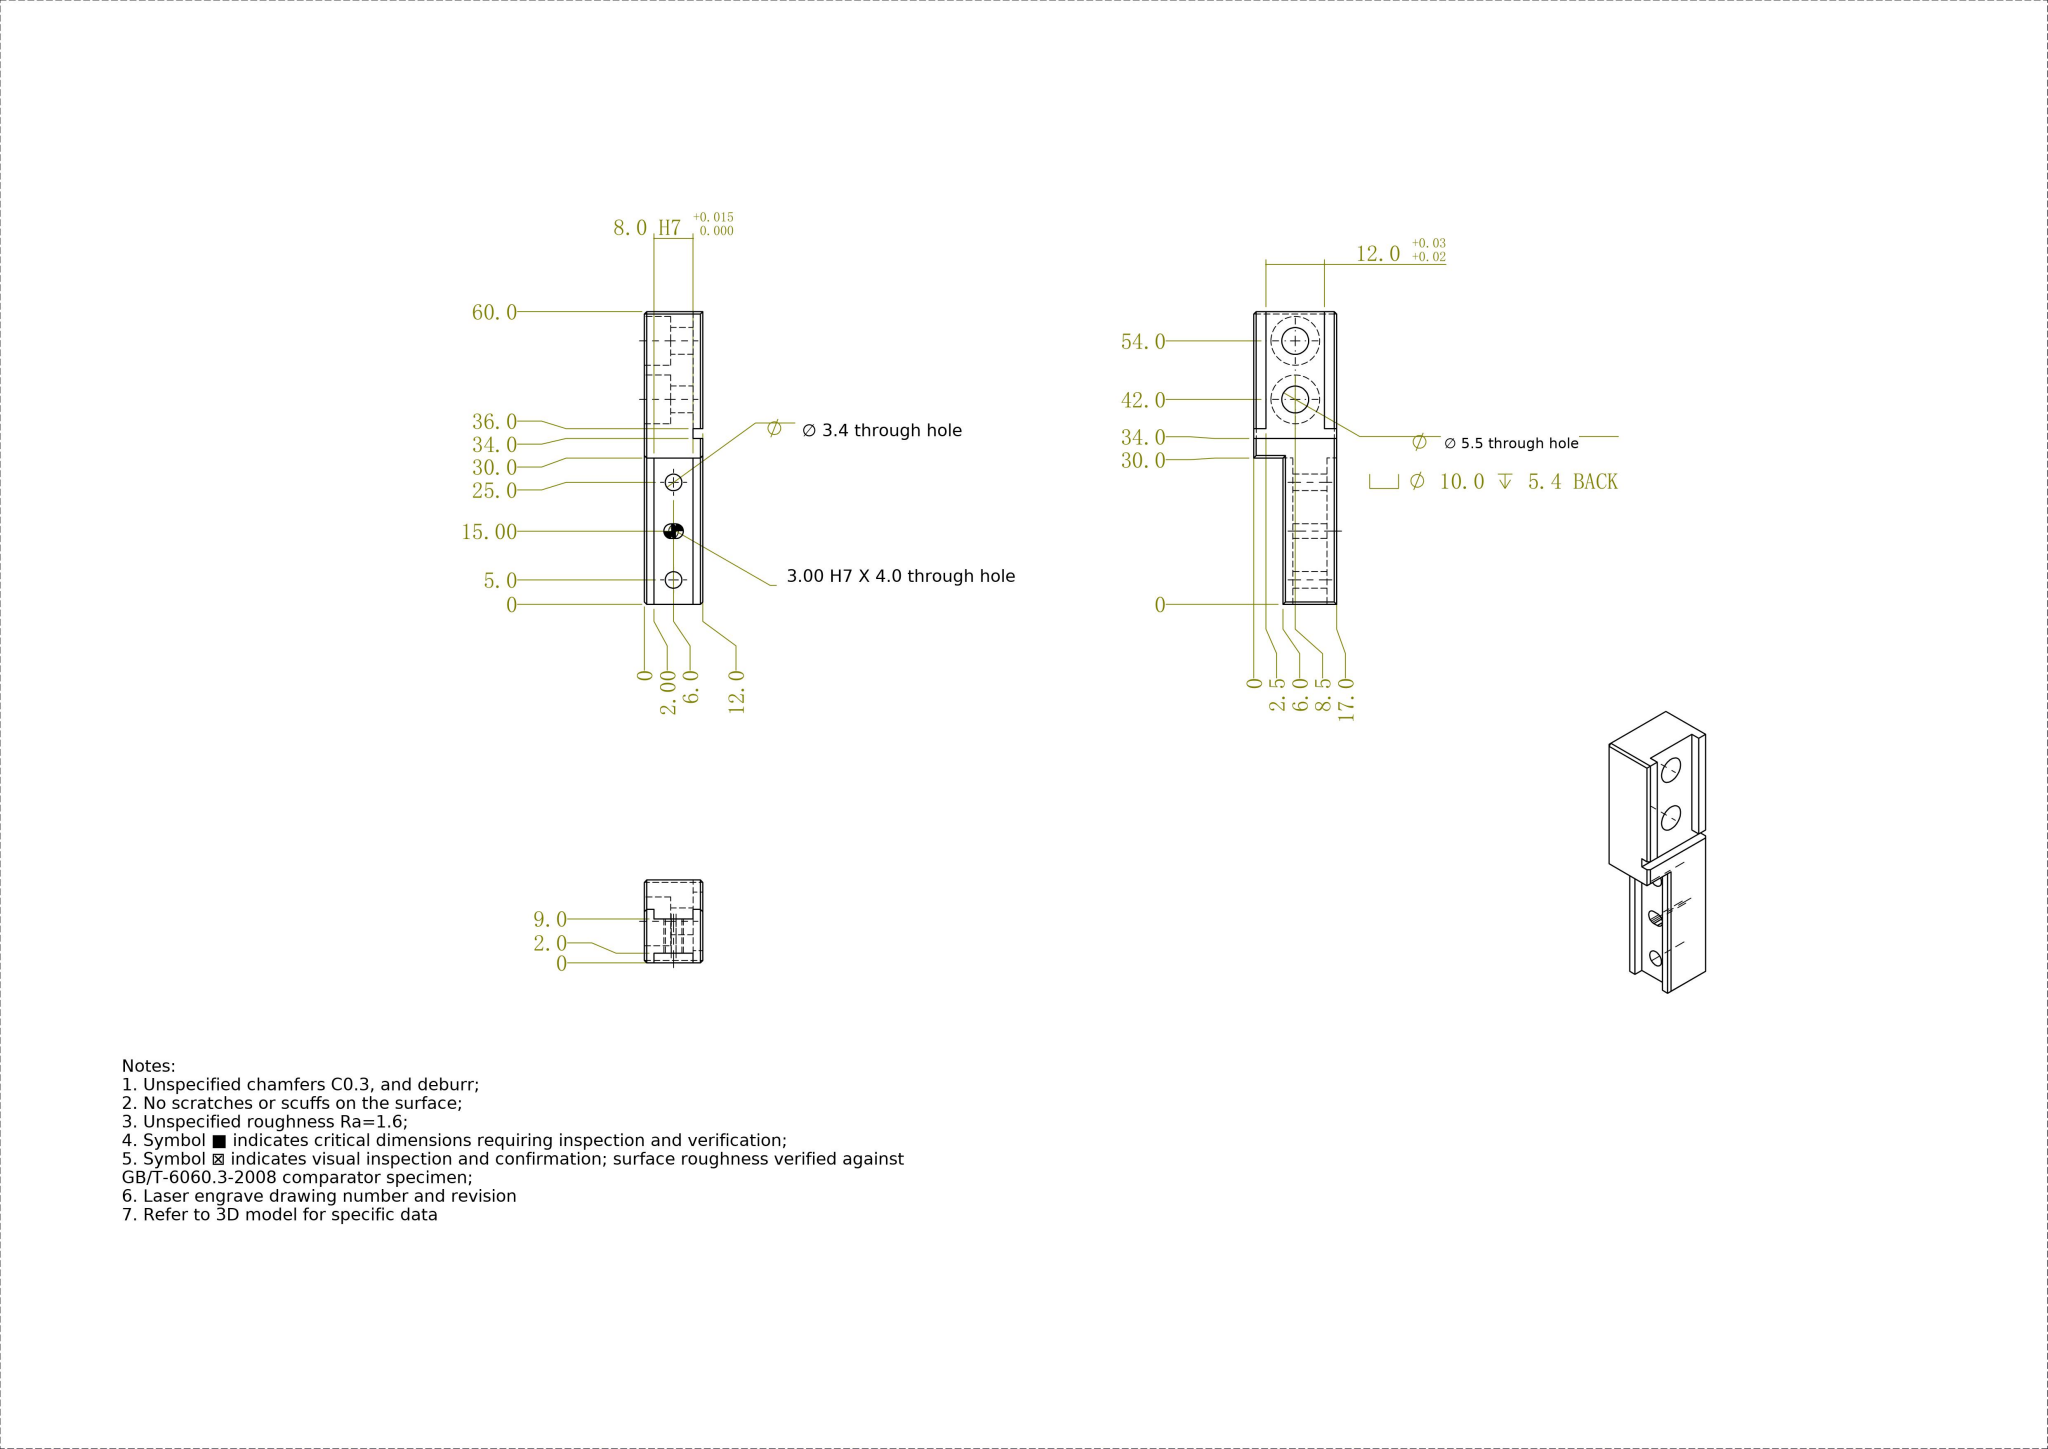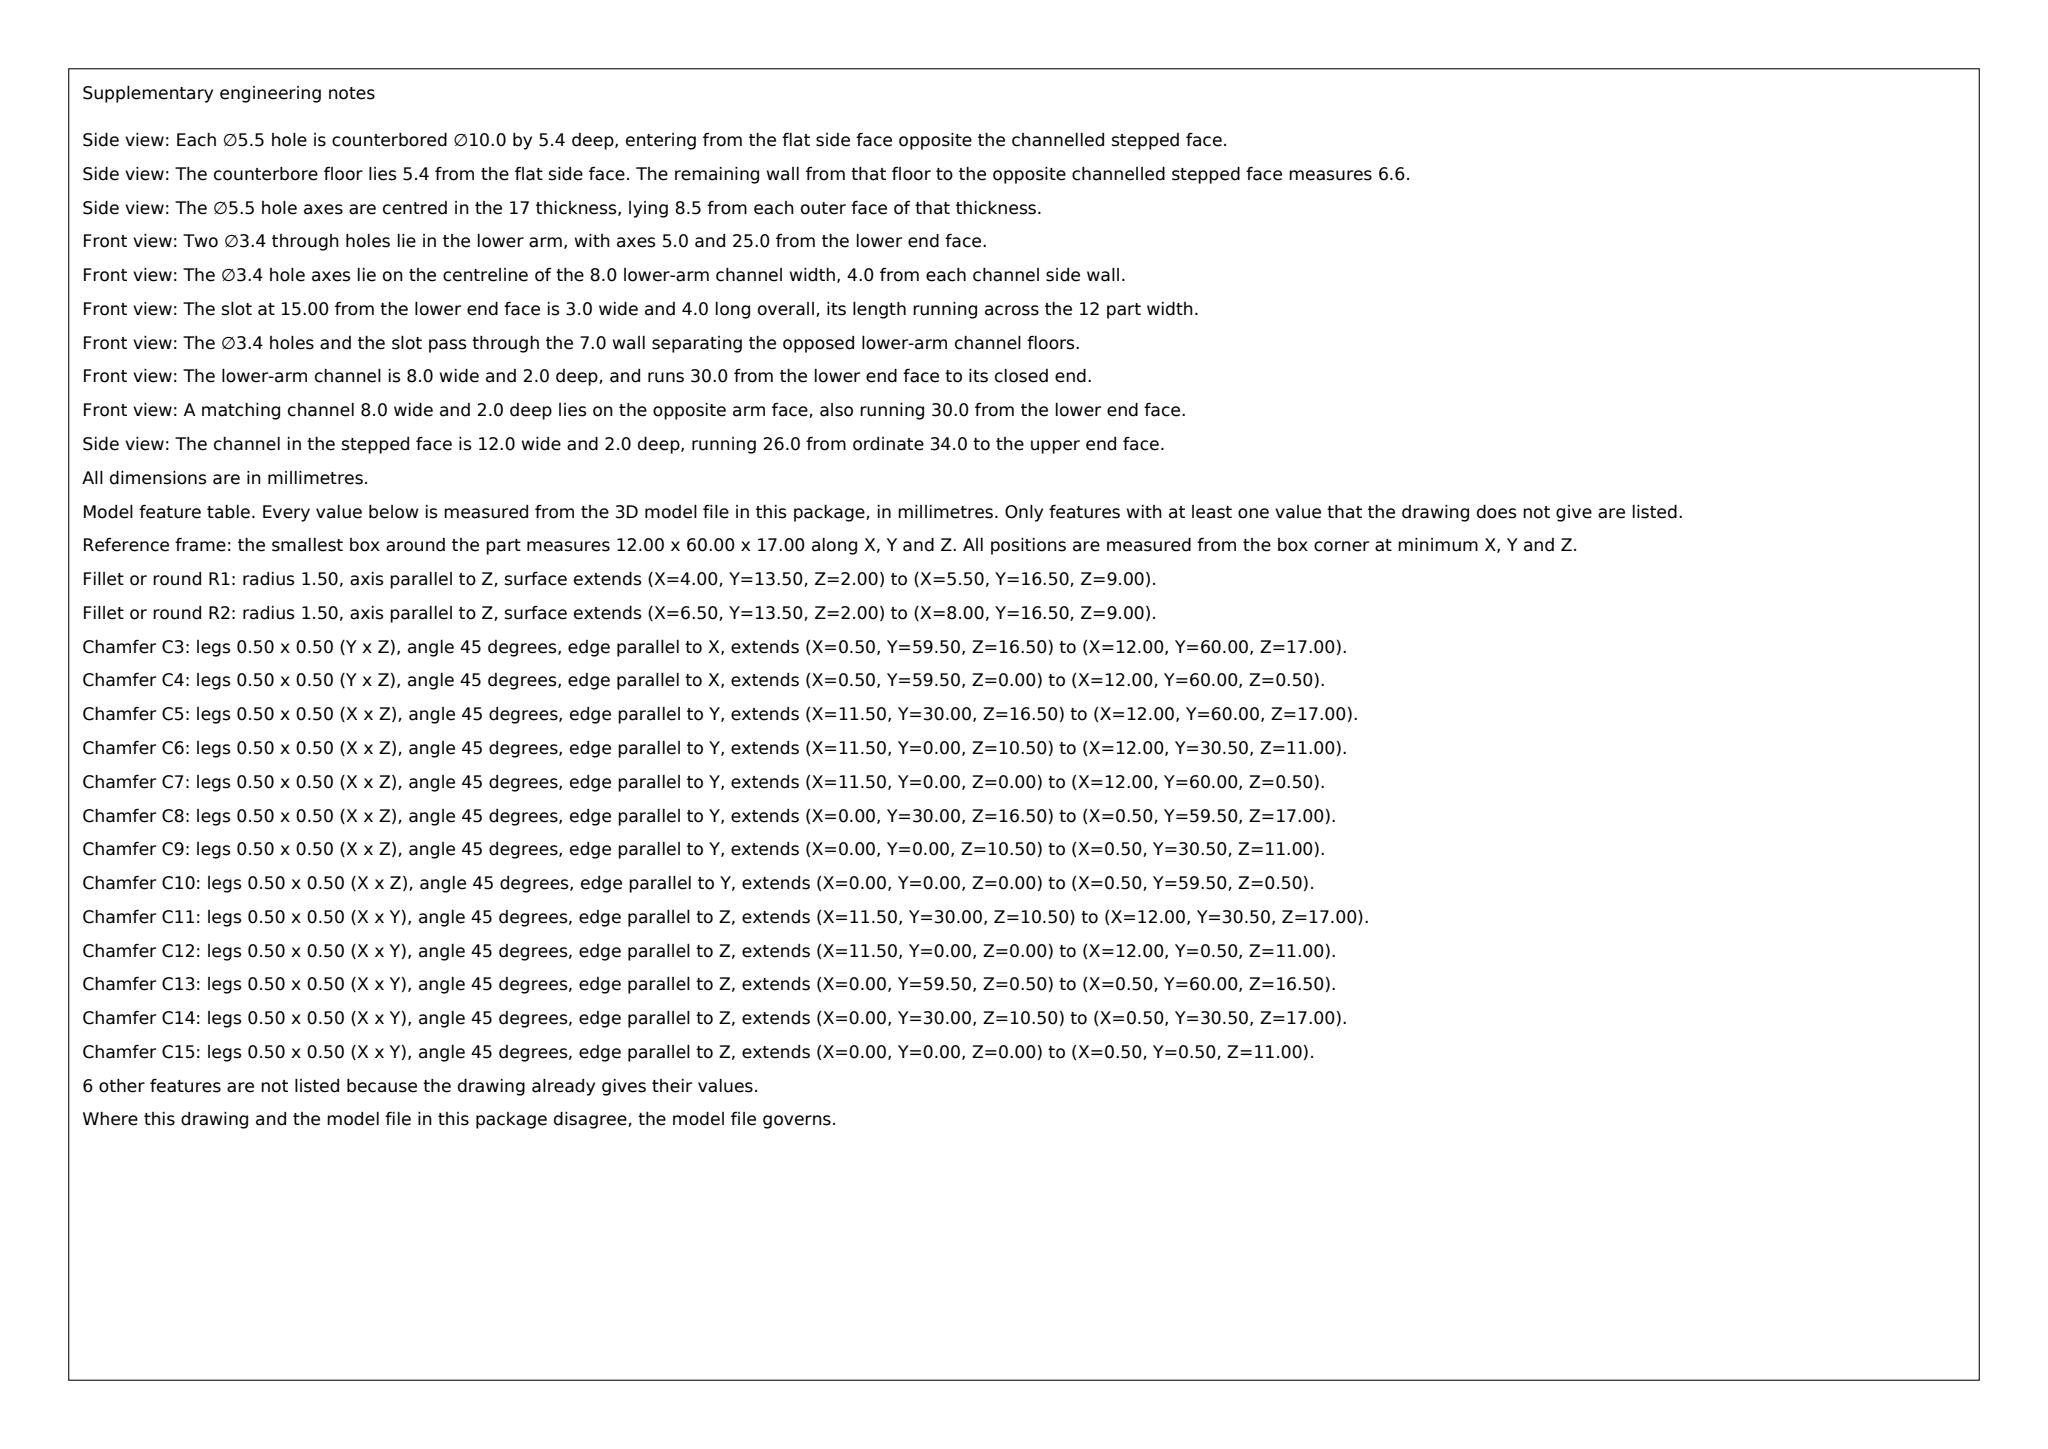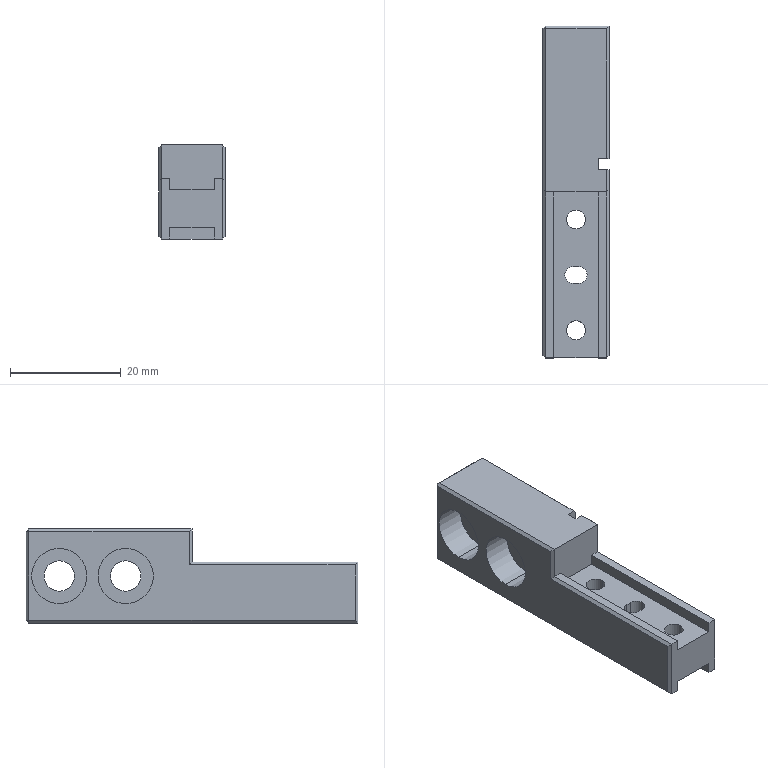Part | SolidWorks | mm | 1 solid | 60 faces | box 12 x 60 x 17 mm | volume 7173 mm3 | plane 45 | cylinder 15 | commonest cylinder face diameters 3.4 x4 10 x4 5.5 x4 3 x3
Drawing notes:
8.0 H7 TOP CHANNEL: FLOOR AT 11.0 FROM 0 DATUM, DP 6.0 FROM 17.0 FACE | from the solid: z-plane 11.0 (x2) with bbox z=17.0; channel width 8.0 H7
SIDE VIEW: UPPER BACK STEP FACES AT 11.0 AND 14.5 FROM 0 DATUM | from the solid: z-planes 11.0 and 14.5 in chain 0/2.5/6.0/8.5/17.0